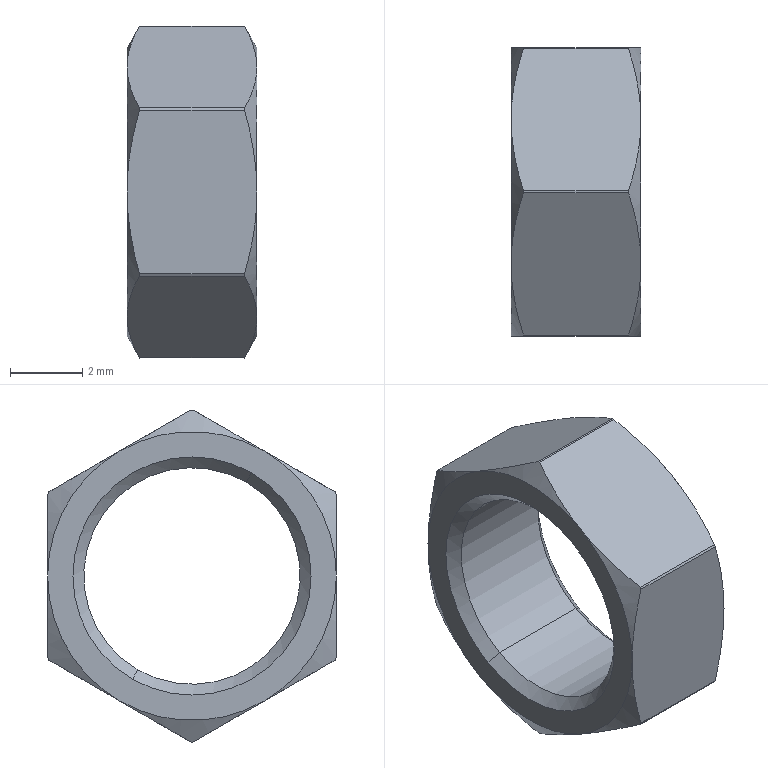Component | SolidWorks | Q1-A12-S21-Q1D.SLDASQ-2_Q1-PACK-SNTRC6-1 | 1 solid | 32 faces | box 3.6 x 8 x 9.2 mm | volume 95 mm3 | cone 16 | cylinder 8 | plane 8 | commonest cylinder face diameters 9.2 x6 6 x2
build123d program:
from build123d import *

# Parameters (mm, degrees)
CUT_EXTRUDE1_DEPTH = 3.6


with BuildPart() as part:
    # Sketch1 → Revolve1 (revolve)
    with BuildSketch(Plane.XY, mode=Mode.PRIVATE) as revolve1_sk:
        Polygon((0, 0), (0, 4), (0.3464, 4.6), (3.254, 4.6), (3.6, 4), (3.6, 0), align=None)
    revolve(revolve1_sk.sketch.rotate(Axis((3.6, 0, 0), (-1, 0, 0)), 270), axis=Axis((3.6, 0, 0), (-1, 0, 0)))

    # Sketch2 → Cut-Extrude1 (cut)
    with BuildSketch(Plane(origin=(0, 0, 0), x_dir=(0, 0, -1), z_dir=(1, 0, 0))):
        Polygon((-8, -4.619), (0, -9.238), (8, -4.619), (8, 4.619), (0, 9.238), (-8, 4.619), align=None)
        Polygon((-4, -2.309), (0, -4.619), (4, -2.309), (4, 2.309), (0, 4.619), (-4, 2.309), align=None, mode=Mode.SUBTRACT)
    extrude(amount=CUT_EXTRUDE1_DEPTH, mode=Mode.SUBTRACT)

    # Sketch3 → Cut-Revolve1 (revolve, cut)
    with BuildSketch(Plane.XY, mode=Mode.PRIVATE) as cut_revolve1_sk:
        Polygon((0, 0), (0, 3.3), (0.3, 3), (3.3, 3), (3.6, 3.3), (3.6, 0), align=None)
    revolve(cut_revolve1_sk.sketch.rotate(Axis((3.6, 0, 0), (-1, 0, 0)), 270), axis=Axis((3.6, 0, 0), (-1, 0, 0)), mode=Mode.SUBTRACT)


solid = part.part

# Placed as in the assembly
solid = solid.moved(Location((1969.5, 0, -156.25), (90, 0, 0)))
STEP:
#1=CARTESIAN_POINT('',(77.669,-0.05906,-6.049));
#2=VERTEX_POINT('',#1);
#3=CARTESIAN_POINT('',(77.669,0.05906,-6.254));
#4=VERTEX_POINT('',#3);
#5=CARTESIAN_POINT('',(77.669,-0.,-6.152));
#6=DIRECTION('',(-1.,-0.,0.));
#7=DIRECTION('',(0.,0.5,-0.866));
#8=AXIS2_PLACEMENT_3D('',#5,#6,#7);
#9=CIRCLE('',#8,0.1181);
#10=EDGE_CURVE('',#2,#4,#9,.T.);
#11=ORIENTED_EDGE('',*,*,#10,.T.);
#12=CARTESIAN_POINT('',(77.681,0.06496,-6.264));
#13=VERTEX_POINT('',#12);
#14=CARTESIAN_POINT('',(77.681,0.06496,-6.264));
#15=DIRECTION('',(0.7071,0.3536,-0.6124));
#16=VECTOR('',#15,39.37);
#17=LINE('',#14,#16);
#18=EDGE_CURVE('',#4,#13,#17,.T.);
#19=ORIENTED_EDGE('',*,*,#18,.T.);
#20=CARTESIAN_POINT('',(77.681,-0.06496,-6.039));
#21=VERTEX_POINT('',#20);
#22=CARTESIAN_POINT('',(77.681,-0.,-6.152));
#23=DIRECTION('',(-1.,-0.,0.));
#24=DIRECTION('',(0.,0.5,-0.866));
#25=AXIS2_PLACEMENT_3D('',#22,#23,#24);
#26=CIRCLE('',#25,0.1299);
#27=EDGE_CURVE('',#21,#13,#26,.T.);
#28=ORIENTED_EDGE('',*,*,#27,.F.);
#29=CARTESIAN_POINT('',(77.681,-0.06496,-6.039));
#30=DIRECTION('',(0.7071,-0.3536,0.6124));
#31=VECTOR('',#30,39.37);
#32=LINE('',#29,#31);
#33=EDGE_CURVE('',#2,#21,#32,.T.);
#34=ORIENTED_EDGE('',*,*,#33,.F.);
#35=EDGE_LOOP('',(#11,#19,#28,#34));
#36=FACE_OUTER_BOUND('',#35,.T.);
#37=CARTESIAN_POINT('',(77.681,-0.,-6.152));
#38=DIRECTION('',(1.,0.,-0.));
#39=DIRECTION('',(0.,-0.5,0.866));
#40=AXIS2_PLACEMENT_3D('',#37,#38,#39);
#41=CONICAL_SURFACE('',#40,0.1299,0.7854);
#42=ADVANCED_FACE('',(#36),#41,.F.);
#43=ORIENTED_EDGE('',*,*,#10,.F.);
#44=CARTESIAN_POINT('',(77.551,-0.05906,-6.049));
#45=VERTEX_POINT('',#44);
#46=CARTESIAN_POINT('',(77.681,-0.05906,-6.049));
#47=DIRECTION('',(-1.,-0.,0.));
#48=VECTOR('',#47,39.37);
#49=LINE('',#46,#48);
#50=EDGE_CURVE('',#2,#45,#49,.T.);
#51=ORIENTED_EDGE('',*,*,#50,.T.);
#52=CARTESIAN_POINT('',(77.551,0.05906,-6.254));
#53=VERTEX_POINT('',#52);
#54=CARTESIAN_POINT('',(77.551,-0.,-6.152));
#55=DIRECTION('',(-1.,-0.,0.));
#56=DIRECTION('',(0.,0.5,-0.866));
#57=AXIS2_PLACEMENT_3D('',#54,#55,#56);
#58=CIRCLE('',#57,0.1181);
#59=EDGE_CURVE('',#45,#53,#58,.T.);
#60=ORIENTED_EDGE('',*,*,#59,.T.);
#61=CARTESIAN_POINT('',(77.681,0.05906,-6.254));
#62=DIRECTION('',(-1.,-0.,0.));
#63=VECTOR('',#62,39.37);
#64=LINE('',#61,#63);
#65=EDGE_CURVE('',#4,#53,#64,.T.);
#66=ORIENTED_EDGE('',*,*,#65,.F.);
#67=EDGE_LOOP('',(#43,#51,#60,#66));
#68=FACE_OUTER_BOUND('',#67,.T.);
#69=CARTESIAN_POINT('',(77.681,-0.,-6.152));
#70=DIRECTION('',(-1.,-0.,0.));
#71=DIRECTION('',(0.,0.5,-0.866));
#72=AXIS2_PLACEMENT_3D('',#69,#70,#71);
#73=CYLINDRICAL_SURFACE('',#72,0.1181);
#74=ADVANCED_FACE('',(#68),#73,.F.);
#75=ORIENTED_EDGE('',*,*,#59,.F.);
#76=CARTESIAN_POINT('',(77.539,-0.06496,-6.039));
#77=VERTEX_POINT('',#76);
#78=CARTESIAN_POINT('',(77.551,-0.05906,-6.049));
#79=DIRECTION('',(-0.7071,-0.3536,0.6124));
#80=VECTOR('',#79,39.37);
#81=LINE('',#78,#80);
#82=EDGE_CURVE('',#45,#77,#81,.T.);
#83=ORIENTED_EDGE('',*,*,#82,.T.);
#84=CARTESIAN_POINT('',(77.539,0.06496,-6.264));
#85=VERTEX_POINT('',#84);
#86=CARTESIAN_POINT('',(77.539,-0.,-6.152));
#87=DIRECTION('',(-1.,-0.,0.));
#88=DIRECTION('',(0.,0.5,-0.866));
#89=AXIS2_PLACEMENT_3D('',#86,#87,#88);
#90=CIRCLE('',#89,0.1299);
#91=EDGE_CURVE('',#77,#85,#90,.T.);
#92=ORIENTED_EDGE('',*,*,#91,.T.);
#93=CARTESIAN_POINT('',(77.551,0.05906,-6.254));
#94=DIRECTION('',(-0.7071,0.3536,-0.6124));
#95=VECTOR('',#94,39.37);
#96=LINE('',#93,#95);
#97=EDGE_CURVE('',#53,#85,#96,.T.);
#98=ORIENTED_EDGE('',*,*,#97,.F.);
#99=EDGE_LOOP('',(#75,#83,#92,#98));
#100=FACE_OUTER_BOUND('',#99,.T.);
#101=CARTESIAN_POINT('',(77.551,-0.,-6.152));
#102=DIRECTION('',(-1.,-0.,0.));
#103=DIRECTION('',(0.,0.5,-0.866));
#104=AXIS2_PLACEMENT_3D('',#101,#102,#103);
#105=CONICAL_SURFACE('',#104,0.1181,0.7854);
#106=ADVANCED_FACE('',(#100),#105,.F.);
#107=CARTESIAN_POINT('',(77.553,0.1575,-6.241));
#108=VERTEX_POINT('',#107);
#109=CARTESIAN_POINT('',(77.553,0.1562,-6.243));
#110=VERTEX_POINT('',#109);
#111=CARTESIAN_POINT('',(77.553,-0.,-6.152));
#112=DIRECTION('',(-1.,-0.,0.));
#113=DIRECTION('',(0.,0.5,-0.866));
#114=AXIS2_PLACEMENT_3D('',#111,#112,#113);
#115=CIRCLE('',#114,0.1811);
#116=EDGE_CURVE('',#108,#110,#115,.T.);
#117=ORIENTED_EDGE('',*,*,#116,.T.);
#118=CARTESIAN_POINT('',(77.539,0.07874,-6.288));
#119=VERTEX_POINT('',#118);
#120=CARTESIAN_POINT('',(77.553,0.1562,-6.243));
#121=CARTESIAN_POINT('',(77.549,0.1436,-6.251));
#122=CARTESIAN_POINT('',(77.545,0.1307,-6.258));
#123=CARTESIAN_POINT('',(77.541,0.1048,-6.273));
#124=CARTESIAN_POINT('',(77.539,0.09182,-6.28));
#125=CARTESIAN_POINT('',(77.539,0.07874,-6.288));
#126=B_SPLINE_CURVE_WITH_KNOTS('',3,(#120,#121,#122,#123,#124,#125),.UNSPECIFIED.,.F.,.F.,(4,2,4),(0.004158,0.005306,0.006455),.UNSPECIFIED.);
#127=EDGE_CURVE('',#110,#119,#126,.T.);
#128=ORIENTED_EDGE('',*,*,#127,.T.);
#129=CARTESIAN_POINT('',(77.539,0.1575,-6.152));
#130=VERTEX_POINT('',#129);
#131=CARTESIAN_POINT('',(77.539,-0.,-6.152));
#132=DIRECTION('',(-1.,-0.,0.));
#133=DIRECTION('',(0.,0.5,-0.866));
#134=AXIS2_PLACEMENT_3D('',#131,#132,#133);
#135=CIRCLE('',#134,0.1575);
#136=EDGE_CURVE('',#130,#119,#135,.T.);
#137=ORIENTED_EDGE('',*,*,#136,.F.);
#138=CARTESIAN_POINT('',(77.539,0.1575,-6.152));
#139=CARTESIAN_POINT('',(77.539,0.1575,-6.167));
#140=CARTESIAN_POINT('',(77.541,0.1575,-6.182));
#141=CARTESIAN_POINT('',(77.545,0.1575,-6.212));
#142=CARTESIAN_POINT('',(77.549,0.1575,-6.226));
#143=CARTESIAN_POINT('',(77.553,0.1575,-6.241));
#144=B_SPLINE_CURVE_WITH_KNOTS('',3,(#138,#139,#140,#141,#142,#143),.UNSPECIFIED.,.F.,.F.,(4,2,4),(0.002298,0.003442,0.004586),.UNSPECIFIED.);
#145=EDGE_CURVE('',#130,#108,#144,.T.);
#146=ORIENTED_EDGE('',*,*,#145,.T.);
#147=EDGE_LOOP('',(#117,#128,#137,#146));
#148=FACE_OUTER_BOUND('',#147,.T.);
#149=CARTESIAN_POINT('',(77.553,-0.,-6.152));
#150=DIRECTION('',(1.,0.,-0.));
#151=DIRECTION('',(0.,-0.5,0.866));
#152=AXIS2_PLACEMENT_3D('',#149,#150,#151);
#153=CONICAL_SURFACE('',#152,0.1811,1.047);
#154=ADVANCED_FACE('',(#148),#153,.T.);
#155=CARTESIAN_POINT('',(77.553,0.1562,-6.06));
#156=VERTEX_POINT('',#155);
#157=CARTESIAN_POINT('',(77.553,0.1575,-6.062));
#158=VERTEX_POINT('',#157);
#159=CARTESIAN_POINT('',(77.553,-0.,-6.152));
#160=DIRECTION('',(-1.,-0.,0.));
#161=DIRECTION('',(0.,0.5,-0.866));
#162=AXIS2_PLACEMENT_3D('',#159,#160,#161);
#163=CIRCLE('',#162,0.1811);
#164=EDGE_CURVE('',#156,#158,#163,.T.);
#165=ORIENTED_EDGE('',*,*,#164,.T.);
#166=CARTESIAN_POINT('',(77.553,0.1575,-6.062));
#167=CARTESIAN_POINT('',(77.545,0.1575,-6.091));
#168=CARTESIAN_POINT('',(77.539,0.1575,-6.121));
#169=CARTESIAN_POINT('',(77.539,0.1575,-6.152));
#170=B_SPLINE_CURVE_WITH_KNOTS('',3,(#166,#167,#168,#169),.UNSPECIFIED.,.F.,.F.,(4,4),(0.00000065,0.002298),.UNSPECIFIED.);
#171=EDGE_CURVE('',#158,#130,#170,.T.);
#172=ORIENTED_EDGE('',*,*,#171,.T.);
#173=CARTESIAN_POINT('',(77.539,0.07874,-6.015));
#174=VERTEX_POINT('',#173);
#175=CARTESIAN_POINT('',(77.539,-0.,-6.152));
#176=DIRECTION('',(-1.,-0.,0.));
#177=DIRECTION('',(0.,0.5,-0.866));
#178=AXIS2_PLACEMENT_3D('',#175,#176,#177);
#179=CIRCLE('',#178,0.1575);
#180=EDGE_CURVE('',#174,#130,#179,.T.);
#181=ORIENTED_EDGE('',*,*,#180,.F.);
#182=CARTESIAN_POINT('',(77.539,0.07874,-6.015));
#183=CARTESIAN_POINT('',(77.539,0.09187,-6.023));
#184=CARTESIAN_POINT('',(77.541,0.105,-6.03));
#185=CARTESIAN_POINT('',(77.545,0.1308,-6.045));
#186=CARTESIAN_POINT('',(77.549,0.1435,-6.053));
#187=CARTESIAN_POINT('',(77.553,0.1562,-6.06));
#188=B_SPLINE_CURVE_WITH_KNOTS('',3,(#182,#183,#184,#185,#186,#187),.UNSPECIFIED.,.F.,.F.,(4,2,4),(0.002298,0.003442,0.004586),.UNSPECIFIED.);
#189=EDGE_CURVE('',#174,#156,#188,.T.);
#190=ORIENTED_EDGE('',*,*,#189,.T.);
#191=EDGE_LOOP('',(#165,#172,#181,#190));
#192=FACE_OUTER_BOUND('',#191,.T.);
#193=CARTESIAN_POINT('',(77.553,-0.,-6.152));
#194=DIRECTION('',(1.,0.,-0.));
#195=DIRECTION('',(0.,-0.5,0.866));
#196=AXIS2_PLACEMENT_3D('',#193,#194,#195);
#197=CONICAL_SURFACE('',#196,0.1811,1.047);
#198=ADVANCED_FACE('',(#192),#197,.T.);
#199=CARTESIAN_POINT('',(77.553,-0.00129,-5.97));
#200=VERTEX_POINT('',#199);
#201=CARTESIAN_POINT('',(77.553,0.00129,-5.97));
#202=VERTEX_POINT('',#201);
#203=CARTESIAN_POINT('',(77.553,-0.,-6.152));
#204=DIRECTION('',(-1.,-0.,0.));
#205=DIRECTION('',(0.,0.5,-0.866));
#206=AXIS2_PLACEMENT_3D('',#203,#204,#205);
#207=CIRCLE('',#206,0.1811);
#208=EDGE_CURVE('',#200,#202,#207,.T.);
#209=ORIENTED_EDGE('',*,*,#208,.T.);
#210=CARTESIAN_POINT('',(77.553,0.00129,-5.97));
#211=CARTESIAN_POINT('',(77.545,0.02665,-5.985));
#212=CARTESIAN_POINT('',(77.539,0.05237,-6.));
#213=CARTESIAN_POINT('',(77.539,0.07874,-6.015));
#214=B_SPLINE_CURVE_WITH_KNOTS('',3,(#210,#211,#212,#213),.UNSPECIFIED.,.F.,.F.,(4,4),(0.00000072,0.002298),.UNSPECIFIED.);
#215=EDGE_CURVE('',#202,#174,#214,.T.);
#216=ORIENTED_EDGE('',*,*,#215,.T.);
#217=CARTESIAN_POINT('',(77.539,-0.07874,-6.015));
#218=VERTEX_POINT('',#217);
#219=CARTESIAN_POINT('',(77.539,-0.,-6.152));
#220=DIRECTION('',(-1.,-0.,0.));
#221=DIRECTION('',(0.,0.5,-0.866));
#222=AXIS2_PLACEMENT_3D('',#219,#220,#221);
#223=CIRCLE('',#222,0.1575);
#224=EDGE_CURVE('',#218,#174,#223,.T.);
#225=ORIENTED_EDGE('',*,*,#224,.F.);
#226=CARTESIAN_POINT('',(77.539,-0.07874,-6.015));
#227=CARTESIAN_POINT('',(77.539,-0.06566,-6.008));
#228=CARTESIAN_POINT('',(77.541,-0.05266,-6.));
#229=CARTESIAN_POINT('',(77.545,-0.0268,-5.985));
#230=CARTESIAN_POINT('',(77.549,-0.0139,-5.978));
#231=CARTESIAN_POINT('',(77.553,-0.00129,-5.97));
#232=B_SPLINE_CURVE_WITH_KNOTS('',3,(#226,#227,#228,#229,#230,#231),.UNSPECIFIED.,.F.,.F.,(4,2,4),(0.004026,0.005172,0.006318),.UNSPECIFIED.);
#233=EDGE_CURVE('',#218,#200,#232,.T.);
#234=ORIENTED_EDGE('',*,*,#233,.T.);
#235=EDGE_LOOP('',(#209,#216,#225,#234));
#236=FACE_OUTER_BOUND('',#235,.T.);
#237=CARTESIAN_POINT('',(77.553,-0.,-6.152));
#238=DIRECTION('',(1.,0.,-0.));
#239=DIRECTION('',(0.,-0.5,0.866));
#240=AXIS2_PLACEMENT_3D('',#237,#238,#239);
#241=CONICAL_SURFACE('',#240,0.1811,1.047);
#242=ADVANCED_FACE('',(#236),#241,.T.);
#243=CARTESIAN_POINT('',(77.553,-0.1575,-6.062));
#244=VERTEX_POINT('',#243);
#245=CARTESIAN_POINT('',(77.553,-0.1562,-6.06));
#246=VERTEX_POINT('',#245);
#247=CARTESIAN_POINT('',(77.553,-0.,-6.152));
#248=DIRECTION('',(-1.,-0.,0.));
#249=DIRECTION('',(0.,0.5,-0.866));
#250=AXIS2_PLACEMENT_3D('',#247,#248,#249);
#251=CIRCLE('',#250,0.1811);
#252=EDGE_CURVE('',#244,#246,#251,.T.);
#253=ORIENTED_EDGE('',*,*,#252,.T.);
#254=CARTESIAN_POINT('',(77.553,-0.1562,-6.06));
#255=CARTESIAN_POINT('',(77.549,-0.1437,-6.053));
#256=CARTESIAN_POINT('',(77.545,-0.131,-6.045));
#257=CARTESIAN_POINT('',(77.541,-0.1051,-6.03));
#258=CARTESIAN_POINT('',(77.539,-0.09183,-6.023));
#259=CARTESIAN_POINT('',(77.539,-0.07874,-6.015));
#260=B_SPLINE_CURVE_WITH_KNOTS('',3,(#254,#255,#256,#257,#258,#259),.UNSPECIFIED.,.F.,.F.,(4,2,4),(0.001734,0.00288,0.004026),.UNSPECIFIED.);
#261=EDGE_CURVE('',#246,#218,#260,.T.);
#262=ORIENTED_EDGE('',*,*,#261,.T.);
#263=CARTESIAN_POINT('',(77.539,-0.1575,-6.152));
#264=VERTEX_POINT('',#263);
#265=CARTESIAN_POINT('',(77.539,-0.,-6.152));
#266=DIRECTION('',(-1.,-0.,0.));
#267=DIRECTION('',(0.,0.5,-0.866));
#268=AXIS2_PLACEMENT_3D('',#265,#266,#267);
#269=CIRCLE('',#268,0.1575);
#270=EDGE_CURVE('',#264,#218,#269,.T.);
#271=ORIENTED_EDGE('',*,*,#270,.F.);
#272=CARTESIAN_POINT('',(77.539,-0.1575,-6.152));
#273=CARTESIAN_POINT('',(77.539,-0.1575,-6.136));
#274=CARTESIAN_POINT('',(77.541,-0.1575,-6.121));
#275=CARTESIAN_POINT('',(77.545,-0.1575,-6.091));
#276=CARTESIAN_POINT('',(77.549,-0.1575,-6.077));
#277=CARTESIAN_POINT('',(77.553,-0.1575,-6.062));
#278=B_SPLINE_CURVE_WITH_KNOTS('',3,(#272,#273,#274,#275,#276,#277),.UNSPECIFIED.,.F.,.F.,(4,2,4),(0.002298,0.003442,0.004586),.UNSPECIFIED.);
#279=EDGE_CURVE('',#264,#244,#278,.T.);
#280=ORIENTED_EDGE('',*,*,#279,.T.);
#281=EDGE_LOOP('',(#253,#262,#271,#280));
#282=FACE_OUTER_BOUND('',#281,.T.);
#283=CARTESIAN_POINT('',(77.553,-0.,-6.152));
#284=DIRECTION('',(1.,0.,-0.));
#285=DIRECTION('',(0.,-0.5,0.866));
#286=AXIS2_PLACEMENT_3D('',#283,#284,#285);
#287=CONICAL_SURFACE('',#286,0.1811,1.047);
#288=ADVANCED_FACE('',(#282),#287,.T.);
#289=CARTESIAN_POINT('',(77.553,-0.1562,-6.243));
#290=VERTEX_POINT('',#289);
#291=CARTESIAN_POINT('',(77.553,-0.1575,-6.241));
#292=VERTEX_POINT('',#291);
#293=CARTESIAN_POINT('',(77.553,-0.,-6.152));
#294=DIRECTION('',(-1.,-0.,0.));
#295=DIRECTION('',(0.,0.5,-0.866));
#296=AXIS2_PLACEMENT_3D('',#293,#294,#295);
#297=CIRCLE('',#296,0.1811);
#298=EDGE_CURVE('',#290,#292,#297,.T.);
#299=ORIENTED_EDGE('',*,*,#298,.T.);
#300=CARTESIAN_POINT('',(77.553,-0.1575,-6.241));
#301=CARTESIAN_POINT('',(77.545,-0.1575,-6.212));
#302=CARTESIAN_POINT('',(77.539,-0.1575,-6.182));
#303=CARTESIAN_POINT('',(77.539,-0.1575,-6.152));
#304=B_SPLINE_CURVE_WITH_KNOTS('',3,(#300,#301,#302,#303),.UNSPECIFIED.,.F.,.F.,(4,4),(0.00000065,0.002298),.UNSPECIFIED.);
#305=EDGE_CURVE('',#292,#264,#304,.T.);
#306=ORIENTED_EDGE('',*,*,#305,.T.);
#307=CARTESIAN_POINT('',(77.539,-0.07874,-6.288));
#308=VERTEX_POINT('',#307);
#309=CARTESIAN_POINT('',(77.539,-0.,-6.152));
#310=DIRECTION('',(-1.,-0.,0.));
#311=DIRECTION('',(0.,0.5,-0.866));
#312=AXIS2_PLACEMENT_3D('',#309,#310,#311);
#313=CIRCLE('',#312,0.1575);
#314=EDGE_CURVE('',#308,#264,#313,.T.);
#315=ORIENTED_EDGE('',*,*,#314,.F.);
#316=CARTESIAN_POINT('',(77.539,-0.07874,-6.288));
#317=CARTESIAN_POINT('',(77.539,-0.09187,-6.28));
#318=CARTESIAN_POINT('',(77.541,-0.105,-6.273));
#319=CARTESIAN_POINT('',(77.545,-0.1308,-6.258));
#320=CARTESIAN_POINT('',(77.549,-0.1435,-6.251));
#321=CARTESIAN_POINT('',(77.553,-0.1562,-6.243));
#322=B_SPLINE_CURVE_WITH_KNOTS('',3,(#316,#317,#318,#319,#320,#321),.UNSPECIFIED.,.F.,.F.,(4,2,4),(0.002298,0.003442,0.004586),.UNSPECIFIED.);
#323=EDGE_CURVE('',#308,#290,#322,.T.);
#324=ORIENTED_EDGE('',*,*,#323,.T.);
#325=EDGE_LOOP('',(#299,#306,#315,#324));
#326=FACE_OUTER_BOUND('',#325,.T.);
#327=CARTESIAN_POINT('',(77.553,-0.,-6.152));
#328=DIRECTION('',(1.,0.,-0.));
#329=DIRECTION('',(0.,-0.5,0.866));
#330=AXIS2_PLACEMENT_3D('',#327,#328,#329);
#331=CONICAL_SURFACE('',#330,0.1811,1.047);
#332=ADVANCED_FACE('',(#326),#331,.T.);
#333=CARTESIAN_POINT('',(77.667,0.1575,-6.241));
#334=VERTEX_POINT('',#333);
#335=CARTESIAN_POINT('',(77.667,0.1562,-6.243));
#336=VERTEX_POINT('',#335);
#337=CARTESIAN_POINT('',(77.667,-0.,-6.152));
#338=DIRECTION('',(-1.,-0.,0.));
#339=DIRECTION('',(0.,0.5,-0.866));
#340=AXIS2_PLACEMENT_3D('',#337,#338,#339);
#341=CIRCLE('',#340,0.1811);
#342=EDGE_CURVE('',#334,#336,#341,.T.);
#343=ORIENTED_EDGE('',*,*,#342,.T.);
#344=CARTESIAN_POINT('',(77.681,0.1562,-6.243));
#345=DIRECTION('',(-1.,-0.,0.));
#346=VECTOR('',#345,39.37);
#347=LINE('',#344,#346);
#348=EDGE_CURVE('',#336,#110,#347,.T.);
#349=ORIENTED_EDGE('',*,*,#348,.T.);
#350=ORIENTED_EDGE('',*,*,#116,.F.);
#351=CARTESIAN_POINT('',(77.681,0.1575,-6.241));
#352=DIRECTION('',(1.,0.,-0.));
#353=VECTOR('',#352,39.37);
#354=LINE('',#351,#353);
#355=EDGE_CURVE('',#108,#334,#354,.T.);
#356=ORIENTED_EDGE('',*,*,#355,.T.);
#357=EDGE_LOOP('',(#343,#349,#350,#356));
#358=FACE_OUTER_BOUND('',#357,.T.);
#359=CARTESIAN_POINT('',(77.681,-0.,-6.152));
#360=DIRECTION('',(-1.,-0.,0.));
#361=DIRECTION('',(0.,0.5,-0.866));
#362=AXIS2_PLACEMENT_3D('',#359,#360,#361);
#363=CYLINDRICAL_SURFACE('',#362,0.1811);
#364=ADVANCED_FACE('',(#358),#363,.T.);
#365=CARTESIAN_POINT('',(77.667,0.1562,-6.06));
#366=VERTEX_POINT('',#365);
#367=CARTESIAN_POINT('',(77.667,0.1575,-6.062));
#368=VERTEX_POINT('',#367);
#369=CARTESIAN_POINT('',(77.667,-0.,-6.152));
#370=DIRECTION('',(-1.,-0.,0.));
#371=DIRECTION('',(0.,0.5,-0.866));
#372=AXIS2_PLACEMENT_3D('',#369,#370,#371);
#373=CIRCLE('',#372,0.1811);
#374=EDGE_CURVE('',#366,#368,#373,.T.);
#375=ORIENTED_EDGE('',*,*,#374,.T.);
#376=CARTESIAN_POINT('',(77.681,0.1575,-6.062));
#377=DIRECTION('',(-1.,-0.,0.));
#378=VECTOR('',#377,39.37);
#379=LINE('',#376,#378);
#380=EDGE_CURVE('',#368,#158,#379,.T.);
#381=ORIENTED_EDGE('',*,*,#380,.T.);
#382=ORIENTED_EDGE('',*,*,#164,.F.);
#383=CARTESIAN_POINT('',(77.681,0.1562,-6.06));
#384=DIRECTION('',(1.,0.,-0.));
#385=VECTOR('',#384,39.37);
#386=LINE('',#383,#385);
#387=EDGE_CURVE('',#156,#366,#386,.T.);
#388=ORIENTED_EDGE('',*,*,#387,.T.);
#389=EDGE_LOOP('',(#375,#381,#382,#388));
#390=FACE_OUTER_BOUND('',#389,.T.);
#391=CARTESIAN_POINT('',(77.681,-0.,-6.152));
#392=DIRECTION('',(-1.,-0.,0.));
#393=DIRECTION('',(0.,0.5,-0.866));
#394=AXIS2_PLACEMENT_3D('',#391,#392,#393);
#395=CYLINDRICAL_SURFACE('',#394,0.1811);
#396=ADVANCED_FACE('',(#390),#395,.T.);
#397=CARTESIAN_POINT('',(77.667,-0.00129,-5.97));
#398=VERTEX_POINT('',#397);
#399=CARTESIAN_POINT('',(77.667,0.00129,-5.97));
#400=VERTEX_POINT('',#399);
#401=CARTESIAN_POINT('',(77.667,-0.,-6.152));
#402=DIRECTION('',(-1.,-0.,0.));
#403=DIRECTION('',(0.,0.5,-0.866));
#404=AXIS2_PLACEMENT_3D('',#401,#402,#403);
#405=CIRCLE('',#404,0.1811);
#406=EDGE_CURVE('',#398,#400,#405,.T.);
#407=ORIENTED_EDGE('',*,*,#406,.T.);
#408=CARTESIAN_POINT('',(77.681,0.00129,-5.97));
#409=DIRECTION('',(-1.,-0.,0.));
#410=VECTOR('',#409,39.37);
#411=LINE('',#408,#410);
#412=EDGE_CURVE('',#400,#202,#411,.T.);
#413=ORIENTED_EDGE('',*,*,#412,.T.);
#414=ORIENTED_EDGE('',*,*,#208,.F.);
#415=CARTESIAN_POINT('',(77.681,-0.00129,-5.97));
#416=DIRECTION('',(1.,0.,-0.));
#417=VECTOR('',#416,39.37);
#418=LINE('',#415,#417);
#419=EDGE_CURVE('',#200,#398,#418,.T.);
#420=ORIENTED_EDGE('',*,*,#419,.T.);
#421=EDGE_LOOP('',(#407,#413,#414,#420));
#422=FACE_OUTER_BOUND('',#421,.T.);
#423=CARTESIAN_POINT('',(77.681,-0.,-6.152));
#424=DIRECTION('',(-1.,-0.,0.));
#425=DIRECTION('',(0.,0.5,-0.866));
#426=AXIS2_PLACEMENT_3D('',#423,#424,#425);
#427=CYLINDRICAL_SURFACE('',#426,0.1811);
#428=ADVANCED_FACE('',(#422),#427,.T.);
#429=CARTESIAN_POINT('',(77.667,-0.1575,-6.062));
#430=VERTEX_POINT('',#429);
#431=CARTESIAN_POINT('',(77.667,-0.1562,-6.06));
#432=VERTEX_POINT('',#431);
#433=CARTESIAN_POINT('',(77.667,-0.,-6.152));
#434=DIRECTION('',(-1.,-0.,0.));
#435=DIRECTION('',(0.,0.5,-0.866));
#436=AXIS2_PLACEMENT_3D('',#433,#434,#435);
#437=CIRCLE('',#436,0.1811);
#438=EDGE_CURVE('',#430,#432,#437,.T.);
#439=ORIENTED_EDGE('',*,*,#438,.T.);
#440=CARTESIAN_POINT('',(77.681,-0.1562,-6.06));
#441=DIRECTION('',(-1.,-0.,0.));
#442=VECTOR('',#441,39.37);
#443=LINE('',#440,#442);
#444=EDGE_CURVE('',#432,#246,#443,.T.);
#445=ORIENTED_EDGE('',*,*,#444,.T.);
#446=ORIENTED_EDGE('',*,*,#252,.F.);
#447=CARTESIAN_POINT('',(77.681,-0.1575,-6.062));
#448=DIRECTION('',(1.,0.,-0.));
#449=VECTOR('',#448,39.37);
#450=LINE('',#447,#449);
#451=EDGE_CURVE('',#244,#430,#450,.T.);
#452=ORIENTED_EDGE('',*,*,#451,.T.);
#453=EDGE_LOOP('',(#439,#445,#446,#452));
#454=FACE_OUTER_BOUND('',#453,.T.);
#455=CARTESIAN_POINT('',(77.681,-0.,-6.152));
#456=DIRECTION('',(-1.,-0.,0.));
#457=DIRECTION('',(0.,0.5,-0.866));
#458=AXIS2_PLACEMENT_3D('',#455,#456,#457);
#459=CYLINDRICAL_SURFACE('',#458,0.1811);
#460=ADVANCED_FACE('',(#454),#459,.T.);
#461=CARTESIAN_POINT('',(77.667,-0.1562,-6.243));
#462=VERTEX_POINT('',#461);
#463=CARTESIAN_POINT('',(77.667,-0.1575,-6.241));
#464=VERTEX_POINT('',#463);
#465=CARTESIAN_POINT('',(77.667,-0.,-6.152));
#466=DIRECTION('',(-1.,-0.,0.));
#467=DIRECTION('',(0.,0.5,-0.866));
#468=AXIS2_PLACEMENT_3D('',#465,#466,#467);
#469=CIRCLE('',#468,0.1811);
#470=EDGE_CURVE('',#462,#464,#469,.T.);
#471=ORIENTED_EDGE('',*,*,#470,.T.);
#472=CARTESIAN_POINT('',(77.681,-0.1575,-6.241));
#473=DIRECTION('',(-1.,-0.,0.));
#474=VECTOR('',#473,39.37);
#475=LINE('',#472,#474);
#476=EDGE_CURVE('',#464,#292,#475,.T.);
#477=ORIENTED_EDGE('',*,*,#476,.T.);
#478=ORIENTED_EDGE('',*,*,#298,.F.);
#479=CARTESIAN_POINT('',(77.681,-0.1562,-6.243));
#480=DIRECTION('',(1.,0.,-0.));
#481=VECTOR('',#480,39.37);
#482=LINE('',#479,#481);
#483=EDGE_CURVE('',#290,#462,#482,.T.);
#484=ORIENTED_EDGE('',*,*,#483,.T.);
#485=EDGE_LOOP('',(#471,#477,#478,#484));
#486=FACE_OUTER_BOUND('',#485,.T.);
#487=CARTESIAN_POINT('',(77.681,-0.,-6.152));
#488=DIRECTION('',(-1.,-0.,0.));
#489=DIRECTION('',(0.,0.5,-0.866));
#490=AXIS2_PLACEMENT_3D('',#487,#488,#489);
#491=CYLINDRICAL_SURFACE('',#490,0.1811);
#492=ADVANCED_FACE('',(#486),#491,.T.);
#493=CARTESIAN_POINT('',(77.667,0.00129,-6.333));
#494=VERTEX_POINT('',#493);
#495=CARTESIAN_POINT('',(77.667,-0.00129,-6.333));
#496=VERTEX_POINT('',#495);
#497=CARTESIAN_POINT('',(77.667,-0.,-6.152));
#498=DIRECTION('',(-1.,-0.,0.));
#499=DIRECTION('',(0.,0.5,-0.866));
#500=AXIS2_PLACEMENT_3D('',#497,#498,#499);
#501=CIRCLE('',#500,0.1811);
#502=EDGE_CURVE('',#494,#496,#501,.T.);
#503=ORIENTED_EDGE('',*,*,#502,.F.);
#504=CARTESIAN_POINT('',(77.681,0.07874,-6.288));
#505=VERTEX_POINT('',#504);
#506=CARTESIAN_POINT('',(77.667,0.00129,-6.333));
#507=CARTESIAN_POINT('',(77.672,0.01382,-6.325));
#508=CARTESIAN_POINT('',(77.675,0.02651,-6.318));
#509=CARTESIAN_POINT('',(77.68,0.05238,-6.303));
#510=CARTESIAN_POINT('',(77.681,0.06565,-6.296));
#511=CARTESIAN_POINT('',(77.681,0.07874,-6.288));
#512=B_SPLINE_CURVE_WITH_KNOTS('',3,(#506,#507,#508,#509,#510,#511),.UNSPECIFIED.,.F.,.F.,(4,2,4),(0.001734,0.00288,0.004026),.UNSPECIFIED.);
#513=EDGE_CURVE('',#494,#505,#512,.T.);
#514=ORIENTED_EDGE('',*,*,#513,.T.);
#515=CARTESIAN_POINT('',(77.681,-0.07874,-6.288));
#516=VERTEX_POINT('',#515);
#517=CARTESIAN_POINT('',(77.681,-0.,-6.152));
#518=DIRECTION('',(-1.,-0.,0.));
#519=DIRECTION('',(0.,0.5,-0.866));
#520=AXIS2_PLACEMENT_3D('',#517,#518,#519);
#521=CIRCLE('',#520,0.1575);
#522=EDGE_CURVE('',#505,#516,#521,.T.);
#523=ORIENTED_EDGE('',*,*,#522,.T.);
#524=CARTESIAN_POINT('',(77.681,-0.07874,-6.288));
#525=CARTESIAN_POINT('',(77.681,-0.06561,-6.296));
#526=CARTESIAN_POINT('',(77.68,-0.05248,-6.303));
#527=CARTESIAN_POINT('',(77.675,-0.02668,-6.318));
#528=CARTESIAN_POINT('',(77.672,-0.01393,-6.325));
#529=CARTESIAN_POINT('',(77.667,-0.00129,-6.333));
#530=B_SPLINE_CURVE_WITH_KNOTS('',3,(#524,#525,#526,#527,#528,#529),.UNSPECIFIED.,.F.,.F.,(4,2,4),(0.002298,0.003442,0.004586),.UNSPECIFIED.);
#531=EDGE_CURVE('',#516,#496,#530,.T.);
#532=ORIENTED_EDGE('',*,*,#531,.T.);
#533=EDGE_LOOP('',(#503,#514,#523,#532));
#534=FACE_OUTER_BOUND('',#533,.T.);
#535=CARTESIAN_POINT('',(77.681,-0.,-6.152));
#536=DIRECTION('',(-1.,-0.,0.));
#537=DIRECTION('',(0.,0.5,-0.866));
#538=AXIS2_PLACEMENT_3D('',#535,#536,#537);
#539=CONICAL_SURFACE('',#538,0.1575,1.047);
#540=ADVANCED_FACE('',(#534),#539,.T.);
#541=CARTESIAN_POINT('',(77.681,0.1575,-6.152));
#542=VERTEX_POINT('',#541);
#543=CARTESIAN_POINT('',(77.681,-0.,-6.152));
#544=DIRECTION('',(-1.,-0.,0.));
#545=DIRECTION('',(0.,0.5,-0.866));
#546=AXIS2_PLACEMENT_3D('',#543,#544,#545);
#547=CIRCLE('',#546,0.1575);
#548=EDGE_CURVE('',#542,#505,#547,.T.);
#549=ORIENTED_EDGE('',*,*,#548,.T.);
#550=CARTESIAN_POINT('',(77.681,0.07874,-6.288));
#551=CARTESIAN_POINT('',(77.681,0.09182,-6.28));
#552=CARTESIAN_POINT('',(77.68,0.1048,-6.273));
#553=CARTESIAN_POINT('',(77.675,0.1307,-6.258));
#554=CARTESIAN_POINT('',(77.672,0.1436,-6.251));
#555=CARTESIAN_POINT('',(77.667,0.1562,-6.243));
#556=B_SPLINE_CURVE_WITH_KNOTS('',3,(#550,#551,#552,#553,#554,#555),.UNSPECIFIED.,.F.,.F.,(4,2,4),(0.004026,0.005172,0.006318),.UNSPECIFIED.);
#557=EDGE_CURVE('',#505,#336,#556,.T.);
#558=ORIENTED_EDGE('',*,*,#557,.T.);
#559=ORIENTED_EDGE('',*,*,#342,.F.);
#560=CARTESIAN_POINT('',(77.667,0.1575,-6.241));
#561=CARTESIAN_POINT('',(77.676,0.1575,-6.212));
#562=CARTESIAN_POINT('',(77.681,0.1575,-6.182));
#563=CARTESIAN_POINT('',(77.681,0.1575,-6.152));
#564=B_SPLINE_CURVE_WITH_KNOTS('',3,(#560,#561,#562,#563),.UNSPECIFIED.,.F.,.F.,(4,4),(0.00000072,0.002298),.UNSPECIFIED.);
#565=EDGE_CURVE('',#334,#542,#564,.T.);
#566=ORIENTED_EDGE('',*,*,#565,.T.);
#567=EDGE_LOOP('',(#549,#558,#559,#566));
#568=FACE_OUTER_BOUND('',#567,.T.);
#569=CARTESIAN_POINT('',(77.681,-0.,-6.152));
#570=DIRECTION('',(-1.,-0.,0.));
#571=DIRECTION('',(0.,0.5,-0.866));
#572=AXIS2_PLACEMENT_3D('',#569,#570,#571);
#573=CONICAL_SURFACE('',#572,0.1575,1.047);
#574=ADVANCED_FACE('',(#568),#573,.T.);
#575=CARTESIAN_POINT('',(77.681,0.07874,-6.015));
#576=VERTEX_POINT('',#575);
#577=CARTESIAN_POINT('',(77.681,-0.,-6.152));
#578=DIRECTION('',(-1.,-0.,0.));
#579=DIRECTION('',(0.,0.5,-0.866));
#580=AXIS2_PLACEMENT_3D('',#577,#578,#579);
#581=CIRCLE('',#580,0.1575);
#582=EDGE_CURVE('',#576,#542,#581,.T.);
#583=ORIENTED_EDGE('',*,*,#582,.T.);
#584=CARTESIAN_POINT('',(77.681,0.1575,-6.152));
#585=CARTESIAN_POINT('',(77.681,0.1575,-6.136));
#586=CARTESIAN_POINT('',(77.68,0.1575,-6.121));
#587=CARTESIAN_POINT('',(77.675,0.1575,-6.091));
#588=CARTESIAN_POINT('',(77.672,0.1575,-6.077));
#589=CARTESIAN_POINT('',(77.667,0.1575,-6.062));
#590=B_SPLINE_CURVE_WITH_KNOTS('',3,(#584,#585,#586,#587,#588,#589),.UNSPECIFIED.,.F.,.F.,(4,2,4),(0.002298,0.003442,0.004586),.UNSPECIFIED.);
#591=EDGE_CURVE('',#542,#368,#590,.T.);
#592=ORIENTED_EDGE('',*,*,#591,.T.);
#593=ORIENTED_EDGE('',*,*,#374,.F.);
#594=CARTESIAN_POINT('',(77.667,0.1562,-6.06));
#595=CARTESIAN_POINT('',(77.676,0.1308,-6.045));
#596=CARTESIAN_POINT('',(77.681,0.1051,-6.03));
#597=CARTESIAN_POINT('',(77.681,0.07874,-6.015));
#598=B_SPLINE_CURVE_WITH_KNOTS('',3,(#594,#595,#596,#597),.UNSPECIFIED.,.F.,.F.,(4,4),(0.00000065,0.002298),.UNSPECIFIED.);
#599=EDGE_CURVE('',#366,#576,#598,.T.);
#600=ORIENTED_EDGE('',*,*,#599,.T.);
#601=EDGE_LOOP('',(#583,#592,#593,#600));
#602=FACE_OUTER_BOUND('',#601,.T.);
#603=CARTESIAN_POINT('',(77.681,-0.,-6.152));
#604=DIRECTION('',(-1.,-0.,0.));
#605=DIRECTION('',(0.,0.5,-0.866));
#606=AXIS2_PLACEMENT_3D('',#603,#604,#605);
#607=CONICAL_SURFACE('',#606,0.1575,1.047);
#608=ADVANCED_FACE('',(#602),#607,.T.);
#609=CARTESIAN_POINT('',(77.681,-0.07874,-6.015));
#610=VERTEX_POINT('',#609);
#611=CARTESIAN_POINT('',(77.681,-0.,-6.152));
#612=DIRECTION('',(-1.,-0.,0.));
#613=DIRECTION('',(0.,0.5,-0.866));
#614=AXIS2_PLACEMENT_3D('',#611,#612,#613);
#615=CIRCLE('',#614,0.1575);
#616=EDGE_CURVE('',#610,#576,#615,.T.);
#617=ORIENTED_EDGE('',*,*,#616,.T.);
#618=CARTESIAN_POINT('',(77.681,0.07874,-6.015));
#619=CARTESIAN_POINT('',(77.681,0.06561,-6.008));
#620=CARTESIAN_POINT('',(77.68,0.05248,-6.));
#621=CARTESIAN_POINT('',(77.675,0.02668,-5.985));
#622=CARTESIAN_POINT('',(77.672,0.01393,-5.978));
#623=CARTESIAN_POINT('',(77.667,0.00129,-5.97));
#624=B_SPLINE_CURVE_WITH_KNOTS('',3,(#618,#619,#620,#621,#622,#623),.UNSPECIFIED.,.F.,.F.,(4,2,4),(0.002298,0.003442,0.004586),.UNSPECIFIED.);
#625=EDGE_CURVE('',#576,#400,#624,.T.);
#626=ORIENTED_EDGE('',*,*,#625,.T.);
#627=ORIENTED_EDGE('',*,*,#406,.F.);
#628=CARTESIAN_POINT('',(77.667,-0.00129,-5.97));
#629=CARTESIAN_POINT('',(77.672,-0.0139,-5.978));
#630=CARTESIAN_POINT('',(77.675,-0.0268,-5.985));
#631=CARTESIAN_POINT('',(77.68,-0.05266,-6.));
#632=CARTESIAN_POINT('',(77.681,-0.06566,-6.008));
#633=CARTESIAN_POINT('',(77.681,-0.07874,-6.015));
#634=B_SPLINE_CURVE_WITH_KNOTS('',3,(#628,#629,#630,#631,#632,#633),.UNSPECIFIED.,.F.,.F.,(4,2,4),(0.004158,0.005306,0.006455),.UNSPECIFIED.);
#635=EDGE_CURVE('',#398,#610,#634,.T.);
#636=ORIENTED_EDGE('',*,*,#635,.T.);
#637=EDGE_LOOP('',(#617,#626,#627,#636));
#638=FACE_OUTER_BOUND('',#637,.T.);
#639=CARTESIAN_POINT('',(77.681,-0.,-6.152));
#640=DIRECTION('',(-1.,-0.,0.));
#641=DIRECTION('',(0.,0.5,-0.866));
#642=AXIS2_PLACEMENT_3D('',#639,#640,#641);
#643=CONICAL_SURFACE('',#642,0.1575,1.047);
#644=ADVANCED_FACE('',(#638),#643,.T.);
#645=CARTESIAN_POINT('',(77.681,-0.1575,-6.152));
#646=VERTEX_POINT('',#645);
#647=CARTESIAN_POINT('',(77.681,-0.,-6.152));
#648=DIRECTION('',(-1.,-0.,0.));
#649=DIRECTION('',(0.,0.5,-0.866));
#650=AXIS2_PLACEMENT_3D('',#647,#648,#649);
#651=CIRCLE('',#650,0.1575);
#652=EDGE_CURVE('',#646,#610,#651,.T.);
#653=ORIENTED_EDGE('',*,*,#652,.T.);
#654=CARTESIAN_POINT('',(77.681,-0.07874,-6.015));
#655=CARTESIAN_POINT('',(77.681,-0.09183,-6.023));
#656=CARTESIAN_POINT('',(77.68,-0.1051,-6.03));
#657=CARTESIAN_POINT('',(77.675,-0.131,-6.045));
#658=CARTESIAN_POINT('',(77.672,-0.1437,-6.053));
#659=CARTESIAN_POINT('',(77.667,-0.1562,-6.06));
#660=B_SPLINE_CURVE_WITH_KNOTS('',3,(#654,#655,#656,#657,#658,#659),.UNSPECIFIED.,.F.,.F.,(4,2,4),(0.006455,0.007604,0.008753),.UNSPECIFIED.);
#661=EDGE_CURVE('',#610,#432,#660,.T.);
#662=ORIENTED_EDGE('',*,*,#661,.T.);
#663=ORIENTED_EDGE('',*,*,#438,.F.);
#664=CARTESIAN_POINT('',(77.667,-0.1575,-6.062));
#665=CARTESIAN_POINT('',(77.676,-0.1575,-6.091));
#666=CARTESIAN_POINT('',(77.681,-0.1575,-6.121));
#667=CARTESIAN_POINT('',(77.681,-0.1575,-6.152));
#668=B_SPLINE_CURVE_WITH_KNOTS('',3,(#664,#665,#666,#667),.UNSPECIFIED.,.F.,.F.,(4,4),(0.00000072,0.002298),.UNSPECIFIED.);
#669=EDGE_CURVE('',#430,#646,#668,.T.);
#670=ORIENTED_EDGE('',*,*,#669,.T.);
#671=EDGE_LOOP('',(#653,#662,#663,#670));
#672=FACE_OUTER_BOUND('',#671,.T.);
#673=CARTESIAN_POINT('',(77.681,-0.,-6.152));
#674=DIRECTION('',(-1.,-0.,0.));
#675=DIRECTION('',(0.,0.5,-0.866));
#676=AXIS2_PLACEMENT_3D('',#673,#674,#675);
#677=CONICAL_SURFACE('',#676,0.1575,1.047);
#678=ADVANCED_FACE('',(#672),#677,.T.);
#679=CARTESIAN_POINT('',(77.539,-0.,-6.152));
#680=DIRECTION('',(-1.,-0.,0.));
#681=DIRECTION('',(0.,0.5,-0.866));
#682=AXIS2_PLACEMENT_3D('',#679,#680,#681);
#683=CIRCLE('',#682,0.1299);
#684=EDGE_CURVE('',#85,#77,#683,.T.);
#685=ORIENTED_EDGE('',*,*,#684,.F.);
#686=ORIENTED_EDGE('',*,*,#91,.F.);
#687=EDGE_LOOP('',(#685,#686));
#688=FACE_BOUND('',#687,.T.);
#689=CARTESIAN_POINT('',(77.539,-0.,-6.152));
#690=DIRECTION('',(-1.,-0.,0.));
#691=DIRECTION('',(0.,0.5,-0.866));
#692=AXIS2_PLACEMENT_3D('',#689,#690,#691);
#693=CIRCLE('',#692,0.1575);
#694=EDGE_CURVE('',#119,#308,#693,.T.);
#695=ORIENTED_EDGE('',*,*,#694,.T.);
#696=ORIENTED_EDGE('',*,*,#314,.T.);
#697=ORIENTED_EDGE('',*,*,#270,.T.);
#698=ORIENTED_EDGE('',*,*,#224,.T.);
#699=ORIENTED_EDGE('',*,*,#180,.T.);
#700=ORIENTED_EDGE('',*,*,#136,.T.);
#701=EDGE_LOOP('',(#695,#696,#697,#698,#699,#700));
#702=FACE_OUTER_BOUND('',#701,.T.);
#703=CARTESIAN_POINT('',(77.539,-0.,-6.152));
#704=DIRECTION('',(1.,0.,-0.));
#705=DIRECTION('',(0.,-0.5,0.866));
#706=AXIS2_PLACEMENT_3D('',#703,#704,#705);
#707=PLANE('',#706);
#708=ADVANCED_FACE('',(#688,#702),#707,.F.);
#709=ORIENTED_EDGE('',*,*,#694,.F.);
#710=CARTESIAN_POINT('',(77.553,0.00129,-6.333));
#711=VERTEX_POINT('',#710);
#712=CARTESIAN_POINT('',(77.539,0.07874,-6.288));
#713=CARTESIAN_POINT('',(77.539,0.06565,-6.296));
#714=CARTESIAN_POINT('',(77.541,0.05238,-6.303));
#715=CARTESIAN_POINT('',(77.545,0.02651,-6.318));
#716=CARTESIAN_POINT('',(77.549,0.01382,-6.325));
#717=CARTESIAN_POINT('',(77.553,0.00129,-6.333));
#718=B_SPLINE_CURVE_WITH_KNOTS('',3,(#712,#713,#714,#715,#716,#717),.UNSPECIFIED.,.F.,.F.,(4,2,4),(0.006455,0.007604,0.008753),.UNSPECIFIED.);
#719=EDGE_CURVE('',#119,#711,#718,.T.);
#720=ORIENTED_EDGE('',*,*,#719,.T.);
#721=CARTESIAN_POINT('',(77.553,-0.00129,-6.333));
#722=VERTEX_POINT('',#721);
#723=CARTESIAN_POINT('',(77.553,-0.,-6.152));
#724=DIRECTION('',(-1.,-0.,0.));
#725=DIRECTION('',(0.,0.5,-0.866));
#726=AXIS2_PLACEMENT_3D('',#723,#724,#725);
#727=CIRCLE('',#726,0.1811);
#728=EDGE_CURVE('',#711,#722,#727,.T.);
#729=ORIENTED_EDGE('',*,*,#728,.T.);
#730=CARTESIAN_POINT('',(77.553,-0.00129,-6.333));
#731=CARTESIAN_POINT('',(77.545,-0.02665,-6.318));
#732=CARTESIAN_POINT('',(77.539,-0.05237,-6.303));
#733=CARTESIAN_POINT('',(77.539,-0.07874,-6.288));
#734=B_SPLINE_CURVE_WITH_KNOTS('',3,(#730,#731,#732,#733),.UNSPECIFIED.,.F.,.F.,(4,4),(0.00000072,0.002298),.UNSPECIFIED.);
#735=EDGE_CURVE('',#722,#308,#734,.T.);
#736=ORIENTED_EDGE('',*,*,#735,.T.);
#737=EDGE_LOOP('',(#709,#720,#729,#736));
#738=FACE_OUTER_BOUND('',#737,.T.);
#739=CARTESIAN_POINT('',(77.553,-0.,-6.152));
#740=DIRECTION('',(1.,0.,-0.));
#741=DIRECTION('',(0.,-0.5,0.866));
#742=AXIS2_PLACEMENT_3D('',#739,#740,#741);
#743=CONICAL_SURFACE('',#742,0.1811,1.047);
#744=ADVANCED_FACE('',(#738),#743,.T.);
#745=ORIENTED_EDGE('',*,*,#728,.F.);
#746=CARTESIAN_POINT('',(77.681,0.00129,-6.333));
#747=DIRECTION('',(1.,0.,-0.));
#748=VECTOR('',#747,39.37);
#749=LINE('',#746,#748);
#750=EDGE_CURVE('',#711,#494,#749,.T.);
#751=ORIENTED_EDGE('',*,*,#750,.T.);
#752=ORIENTED_EDGE('',*,*,#502,.T.);
#753=CARTESIAN_POINT('',(77.681,-0.00129,-6.333));
#754=DIRECTION('',(-1.,-0.,0.));
#755=VECTOR('',#754,39.37);
#756=LINE('',#753,#755);
#757=EDGE_CURVE('',#496,#722,#756,.T.);
#758=ORIENTED_EDGE('',*,*,#757,.T.);
#759=EDGE_LOOP('',(#745,#751,#752,#758));
#760=FACE_OUTER_BOUND('',#759,.T.);
#761=CARTESIAN_POINT('',(77.681,-0.,-6.152));
#762=DIRECTION('',(-1.,-0.,0.));
#763=DIRECTION('',(0.,0.5,-0.866));
#764=AXIS2_PLACEMENT_3D('',#761,#762,#763);
#765=CYLINDRICAL_SURFACE('',#764,0.1811);
#766=ADVANCED_FACE('',(#760),#765,.T.);
#767=CARTESIAN_POINT('',(77.681,-0.,-6.152));
#768=DIRECTION('',(-1.,-0.,0.));
#769=DIRECTION('',(0.,0.5,-0.866));
#770=AXIS2_PLACEMENT_3D('',#767,#768,#769);
#771=CIRCLE('',#770,0.1575);
#772=EDGE_CURVE('',#516,#646,#771,.T.);
#773=ORIENTED_EDGE('',*,*,#772,.T.);
#774=CARTESIAN_POINT('',(77.681,-0.1575,-6.152));
#775=CARTESIAN_POINT('',(77.681,-0.1575,-6.167));
#776=CARTESIAN_POINT('',(77.68,-0.1575,-6.182));
#777=CARTESIAN_POINT('',(77.675,-0.1575,-6.212));
#778=CARTESIAN_POINT('',(77.672,-0.1575,-6.226));
#779=CARTESIAN_POINT('',(77.667,-0.1575,-6.241));
#780=B_SPLINE_CURVE_WITH_KNOTS('',3,(#774,#775,#776,#777,#778,#779),.UNSPECIFIED.,.F.,.F.,(4,2,4),(0.002298,0.003442,0.004586),.UNSPECIFIED.);
#781=EDGE_CURVE('',#646,#464,#780,.T.);
#782=ORIENTED_EDGE('',*,*,#781,.T.);
#783=ORIENTED_EDGE('',*,*,#470,.F.);
#784=CARTESIAN_POINT('',(77.667,-0.1562,-6.243));
#785=CARTESIAN_POINT('',(77.676,-0.1308,-6.258));
#786=CARTESIAN_POINT('',(77.681,-0.1051,-6.273));
#787=CARTESIAN_POINT('',(77.681,-0.07874,-6.288));
#788=B_SPLINE_CURVE_WITH_KNOTS('',3,(#784,#785,#786,#787),.UNSPECIFIED.,.F.,.F.,(4,4),(0.00000065,0.002298),.UNSPECIFIED.);
#789=EDGE_CURVE('',#462,#516,#788,.T.);
#790=ORIENTED_EDGE('',*,*,#789,.T.);
#791=EDGE_LOOP('',(#773,#782,#783,#790));
#792=FACE_OUTER_BOUND('',#791,.T.);
#793=CARTESIAN_POINT('',(77.681,-0.,-6.152));
#794=DIRECTION('',(-1.,-0.,0.));
#795=DIRECTION('',(0.,0.5,-0.866));
#796=AXIS2_PLACEMENT_3D('',#793,#794,#795);
#797=CONICAL_SURFACE('',#796,0.1575,1.047);
#798=ADVANCED_FACE('',(#792),#797,.T.);
#799=ORIENTED_EDGE('',*,*,#27,.T.);
#800=CARTESIAN_POINT('',(77.681,-0.,-6.152));
#801=DIRECTION('',(-1.,-0.,0.));
#802=DIRECTION('',(0.,0.5,-0.866));
#803=AXIS2_PLACEMENT_3D('',#800,#801,#802);
#804=CIRCLE('',#803,0.1299);
#805=EDGE_CURVE('',#13,#21,#804,.T.);
#806=ORIENTED_EDGE('',*,*,#805,.T.);
#807=EDGE_LOOP('',(#799,#806));
#808=FACE_BOUND('',#807,.T.);
#809=ORIENTED_EDGE('',*,*,#522,.F.);
#810=ORIENTED_EDGE('',*,*,#548,.F.);
#811=ORIENTED_EDGE('',*,*,#582,.F.);
#812=ORIENTED_EDGE('',*,*,#616,.F.);
#813=ORIENTED_EDGE('',*,*,#652,.F.);
#814=ORIENTED_EDGE('',*,*,#772,.F.);
#815=EDGE_LOOP('',(#809,#810,#811,#812,#813,#814));
#816=FACE_OUTER_BOUND('',#815,.T.);
#817=CARTESIAN_POINT('',(77.681,-0.1364,-6.23));
#818=DIRECTION('',(-1.,-0.,0.));
#819=DIRECTION('',(-0.,0.5,-0.866));
#820=AXIS2_PLACEMENT_3D('',#817,#818,#819);
#821=PLANE('',#820);
#822=ADVANCED_FACE('',(#808,#816),#821,.F.);
#823=ORIENTED_EDGE('',*,*,#757,.F.);
#824=ORIENTED_EDGE('',*,*,#531,.F.);
#825=ORIENTED_EDGE('',*,*,#789,.F.);
#826=ORIENTED_EDGE('',*,*,#483,.F.);
#827=ORIENTED_EDGE('',*,*,#323,.F.);
#828=ORIENTED_EDGE('',*,*,#735,.F.);
#829=EDGE_LOOP('',(#823,#824,#825,#826,#827,#828));
#830=FACE_OUTER_BOUND('',#829,.T.);
#831=CARTESIAN_POINT('',(77.681,-0.1575,-6.242));
#832=DIRECTION('',(0.,0.5,0.866));
#833=DIRECTION('',(0.,-0.866,0.5));
#834=AXIS2_PLACEMENT_3D('',#831,#832,#833);
#835=PLANE('',#834);
#836=ADVANCED_FACE('',(#830),#835,.F.);
#837=ORIENTED_EDGE('',*,*,#476,.F.);
#838=ORIENTED_EDGE('',*,*,#781,.F.);
#839=ORIENTED_EDGE('',*,*,#669,.F.);
#840=ORIENTED_EDGE('',*,*,#451,.F.);
#841=ORIENTED_EDGE('',*,*,#279,.F.);
#842=ORIENTED_EDGE('',*,*,#305,.F.);
#843=EDGE_LOOP('',(#837,#838,#839,#840,#841,#842));
#844=FACE_OUTER_BOUND('',#843,.T.);
#845=CARTESIAN_POINT('',(77.681,-0.1575,-6.061));
#846=DIRECTION('',(-0.,1.,-0.));
#847=DIRECTION('',(0.,0.,1.));
#848=AXIS2_PLACEMENT_3D('',#845,#846,#847);
#849=PLANE('',#848);
#850=ADVANCED_FACE('',(#844),#849,.F.);
#851=ORIENTED_EDGE('',*,*,#444,.F.);
#852=ORIENTED_EDGE('',*,*,#661,.F.);
#853=ORIENTED_EDGE('',*,*,#635,.F.);
#854=ORIENTED_EDGE('',*,*,#419,.F.);
#855=ORIENTED_EDGE('',*,*,#233,.F.);
#856=ORIENTED_EDGE('',*,*,#261,.F.);
#857=EDGE_LOOP('',(#851,#852,#853,#854,#855,#856));
#858=FACE_OUTER_BOUND('',#857,.T.);
#859=CARTESIAN_POINT('',(77.681,0.,-5.97));
#860=DIRECTION('',(-0.,0.5,-0.866));
#861=DIRECTION('',(1.,0.,-0.));
#862=AXIS2_PLACEMENT_3D('',#859,#860,#861);
#863=PLANE('',#862);
#864=ADVANCED_FACE('',(#858),#863,.F.);
#865=ORIENTED_EDGE('',*,*,#412,.F.);
#866=ORIENTED_EDGE('',*,*,#625,.F.);
#867=ORIENTED_EDGE('',*,*,#599,.F.);
#868=ORIENTED_EDGE('',*,*,#387,.F.);
#869=ORIENTED_EDGE('',*,*,#189,.F.);
#870=ORIENTED_EDGE('',*,*,#215,.F.);
#871=EDGE_LOOP('',(#865,#866,#867,#868,#869,#870));
#872=FACE_OUTER_BOUND('',#871,.T.);
#873=CARTESIAN_POINT('',(77.681,0.1575,-6.061));
#874=DIRECTION('',(-0.,-0.5,-0.866));
#875=DIRECTION('',(-0.,0.866,-0.5));
#876=AXIS2_PLACEMENT_3D('',#873,#874,#875);
#877=PLANE('',#876);
#878=ADVANCED_FACE('',(#872),#877,.F.);
#879=ORIENTED_EDGE('',*,*,#380,.F.);
#880=ORIENTED_EDGE('',*,*,#591,.F.);
#881=ORIENTED_EDGE('',*,*,#565,.F.);
#882=ORIENTED_EDGE('',*,*,#355,.F.);
#883=ORIENTED_EDGE('',*,*,#145,.F.);
#884=ORIENTED_EDGE('',*,*,#171,.F.);
#885=EDGE_LOOP('',(#879,#880,#881,#882,#883,#884));
#886=FACE_OUTER_BOUND('',#885,.T.);
#887=CARTESIAN_POINT('',(77.681,0.1575,-6.242));
#888=DIRECTION('',(0.,-1.,0.));
#889=DIRECTION('',(-0.,-0.,-1.));
#890=AXIS2_PLACEMENT_3D('',#887,#888,#889);
#891=PLANE('',#890);
#892=ADVANCED_FACE('',(#886),#891,.F.);
#893=ORIENTED_EDGE('',*,*,#348,.F.);
#894=ORIENTED_EDGE('',*,*,#557,.F.);
#895=ORIENTED_EDGE('',*,*,#513,.F.);
#896=ORIENTED_EDGE('',*,*,#750,.F.);
#897=ORIENTED_EDGE('',*,*,#719,.F.);
#898=ORIENTED_EDGE('',*,*,#127,.F.);
#899=EDGE_LOOP('',(#893,#894,#895,#896,#897,#898));
#900=FACE_OUTER_BOUND('',#899,.T.);
#901=CARTESIAN_POINT('',(77.681,-0.,-6.333));
#902=DIRECTION('',(0.,-0.5,0.866));
#903=DIRECTION('',(-1.,-0.,0.));
#904=AXIS2_PLACEMENT_3D('',#901,#902,#903);
#905=PLANE('',#904);
#906=ADVANCED_FACE('',(#900),#905,.F.);
#907=ORIENTED_EDGE('',*,*,#82,.F.);
#908=CARTESIAN_POINT('',(77.551,-0.,-6.152));
#909=DIRECTION('',(-1.,-0.,0.));
#910=DIRECTION('',(0.,0.5,-0.866));
#911=AXIS2_PLACEMENT_3D('',#908,#909,#910);
#912=CIRCLE('',#911,0.1181);
#913=EDGE_CURVE('',#53,#45,#912,.T.);
#914=ORIENTED_EDGE('',*,*,#913,.F.);
#915=ORIENTED_EDGE('',*,*,#97,.T.);
#916=ORIENTED_EDGE('',*,*,#684,.T.);
#917=EDGE_LOOP('',(#907,#914,#915,#916));
#918=FACE_OUTER_BOUND('',#917,.T.);
#919=CARTESIAN_POINT('',(77.551,-0.,-6.152));
#920=DIRECTION('',(-1.,-0.,0.));
#921=DIRECTION('',(0.,0.5,-0.866));
#922=AXIS2_PLACEMENT_3D('',#919,#920,#921);
#923=CONICAL_SURFACE('',#922,0.1181,0.7854);
#924=ADVANCED_FACE('',(#918),#923,.F.);
#925=ORIENTED_EDGE('',*,*,#50,.F.);
#926=CARTESIAN_POINT('',(77.669,-0.,-6.152));
#927=DIRECTION('',(-1.,-0.,0.));
#928=DIRECTION('',(0.,0.5,-0.866));
#929=AXIS2_PLACEMENT_3D('',#926,#927,#928);
#930=CIRCLE('',#929,0.1181);
#931=EDGE_CURVE('',#4,#2,#930,.T.);
#932=ORIENTED_EDGE('',*,*,#931,.F.);
#933=ORIENTED_EDGE('',*,*,#65,.T.);
#934=ORIENTED_EDGE('',*,*,#913,.T.);
#935=EDGE_LOOP('',(#925,#932,#933,#934));
#936=FACE_OUTER_BOUND('',#935,.T.);
#937=CARTESIAN_POINT('',(77.681,-0.,-6.152));
#938=DIRECTION('',(-1.,-0.,0.));
#939=DIRECTION('',(0.,0.5,-0.866));
#940=AXIS2_PLACEMENT_3D('',#937,#938,#939);
#941=CYLINDRICAL_SURFACE('',#940,0.1181);
#942=ADVANCED_FACE('',(#936),#941,.F.);
#943=ORIENTED_EDGE('',*,*,#18,.F.);
#944=ORIENTED_EDGE('',*,*,#931,.T.);
#945=ORIENTED_EDGE('',*,*,#33,.T.);
#946=ORIENTED_EDGE('',*,*,#805,.F.);
#947=EDGE_LOOP('',(#943,#944,#945,#946));
#948=FACE_OUTER_BOUND('',#947,.T.);
#949=CARTESIAN_POINT('',(77.681,-0.,-6.152));
#950=DIRECTION('',(1.,0.,-0.));
#951=DIRECTION('',(0.,-0.5,0.866));
#952=AXIS2_PLACEMENT_3D('',#949,#950,#951);
#953=CONICAL_SURFACE('',#952,0.1299,0.7854);
#954=ADVANCED_FACE('',(#948),#953,.F.);
#955=CLOSED_SHELL('',(#42,#74,#106,#154,#198,#242,#288,#332,#364,#396,#428,#460,#492,#540,#574,#608,#644,#678,#708,#744,#766,#798,#822,#836,#850,#864,#878,#892,#906,#924,#942,#954));
#956=MANIFOLD_SOLID_BREP('',#955);
#957=CARTESIAN_POINT('',(0.,0.,0.));
#958=DIRECTION('',(0.,0.,1.));
#959=DIRECTION('',(1.,0.,0.));
#960=AXIS2_PLACEMENT_3D('',#957,#958,#959);
#961=(LENGTH_UNIT()NAMED_UNIT(*)SI_UNIT($,.METRE.));
#962=LENGTH_MEASURE_WITH_UNIT(LENGTH_MEASURE(0.0254),#961);
#963=DIMENSIONAL_EXPONENTS(1.,0.,0.,0.,0.,0.,0.);
#964=(CONVERSION_BASED_UNIT('',#962)LENGTH_UNIT()NAMED_UNIT(#963));
#965=UNCERTAINTY_MEASURE_WITH_UNIT(LENGTH_MEASURE(0.00001),#964,'','');
#966=(NAMED_UNIT(*)PLANE_ANGLE_UNIT()SI_UNIT($,.RADIAN.));
#967=(NAMED_UNIT(*)SI_UNIT($,.STERADIAN.)SOLID_ANGLE_UNIT());
#968=(GEOMETRIC_REPRESENTATION_CONTEXT(3)GLOBAL_UNCERTAINTY_ASSIGNED_CONTEXT((#965))GLOBAL_UNIT_ASSIGNED_CONTEXT((#964,#966,#967))REPRESENTATION_CONTEXT('',''));
#969=ADVANCED_BREP_SHAPE_REPRESENTATION('',(#956,#960),#968);
#970=COLOUR_RGB('',0.7922,0.8196,0.9333);
#971=FILL_AREA_STYLE_COLOUR('',#970);
#972=FILL_AREA_STYLE('',(#971));
#973=SURFACE_STYLE_FILL_AREA(#972);
#974=SURFACE_SIDE_STYLE('',(#973));
#975=SURFACE_STYLE_USAGE(.BOTH.,#974);
#976=PRESENTATION_STYLE_ASSIGNMENT((#975));
#977=STYLED_ITEM('',(#976),#956);
#978=PRESENTATION_LAYER_ASSIGNMENT('','',(#977));
#979=(LENGTH_UNIT()NAMED_UNIT(*)SI_UNIT($,.METRE.));
#980=LENGTH_MEASURE_WITH_UNIT(LENGTH_MEASURE(0.0254),#979);
#981=DIMENSIONAL_EXPONENTS(1.,0.,0.,0.,0.,0.,0.);
#982=(CONVERSION_BASED_UNIT('',#980)LENGTH_UNIT()NAMED_UNIT(#981));
#983=UNCERTAINTY_MEASURE_WITH_UNIT(LENGTH_MEASURE(0.00001),#982,'','');
#984=(NAMED_UNIT(*)PLANE_ANGLE_UNIT()SI_UNIT($,.RADIAN.));
#985=(NAMED_UNIT(*)SI_UNIT($,.STERADIAN.)SOLID_ANGLE_UNIT());
#986=(GEOMETRIC_REPRESENTATION_CONTEXT(3)GLOBAL_UNCERTAINTY_ASSIGNED_CONTEXT((#983))GLOBAL_UNIT_ASSIGNED_CONTEXT((#982,#984,#985))REPRESENTATION_CONTEXT('',''));
#987=MECHANICAL_DESIGN_GEOMETRIC_PRESENTATION_REPRESENTATION('',(#977),#986);